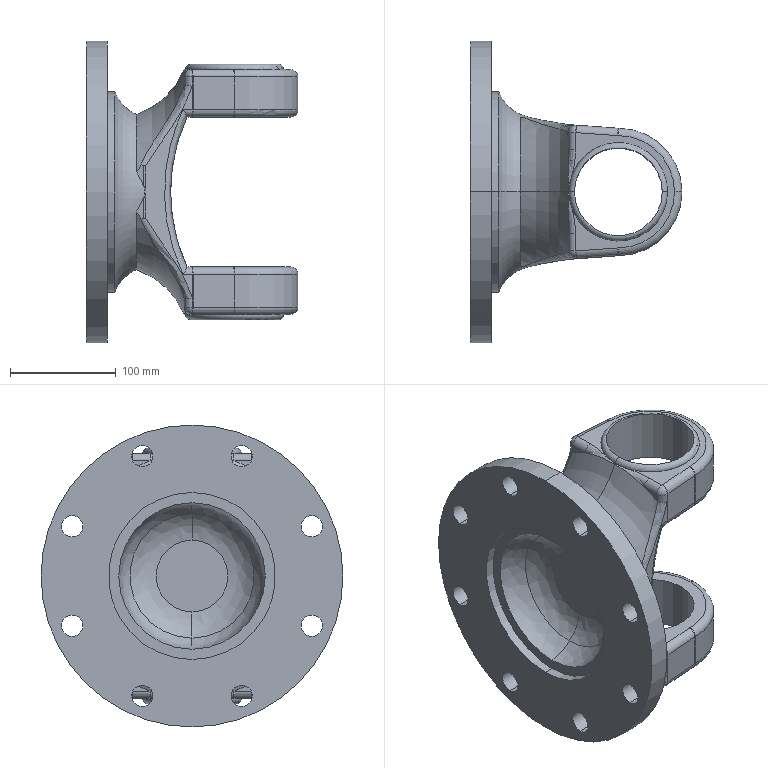Component | NX | BRIDA_587_PREDETERMINADO_COMO_MECANIZADA | 1 solid | 151 faces | volume 2601224 mm3 | cylinder 63 | torus 40 | plane 26 | spline 18 | sphere 4 | commonest cylinder face diameters 14 x28 20.1 x16 83 x4 120 x4 157.541 x2 285 x2 188.837 x2 508.663 x2